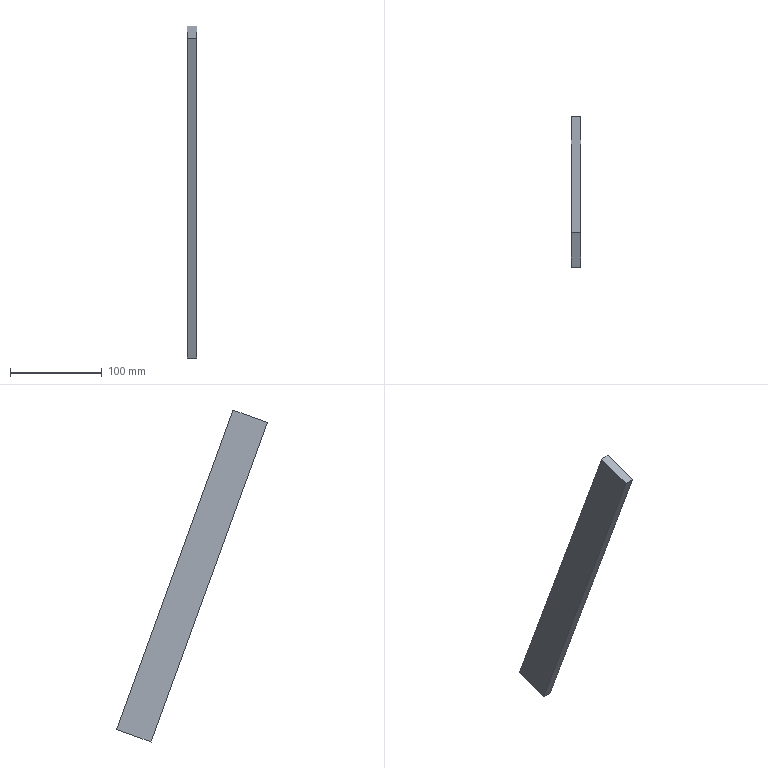Component | SolidWorks | Rebro sipke-2-34 | 1 solid | 6 faces | box 10 x 164.17 x 361.36 mm | volume 148000 mm3 | plane 6
build123d program:
from build123d import *

# Parameters (mm, degrees)
BOSS_EXTRUDE1_DEPTH = 10


with BuildPart() as part:
    # Sketch1 → Boss-Extrude1 (new body)
    with BuildSketch(Plane.XY):
        Polygon((-494.224, -762.65), (-530.101, -744.961), (-366.483, -413.104), (-330.606, -430.793), align=None)
    extrude(amount=-BOSS_EXTRUDE1_DEPTH)


solid = part.part

# Placed as in the assembly
solid = solid.moved(Location((16.4, -1316.705, 597.79), (83.762, -90, 0)))
STEP:
#1=COLOUR_RGB('',0.7922,0.8196,0.9333);
#2=FILL_AREA_STYLE_COLOUR('',#1);
#3=FILL_AREA_STYLE('',(#2));
#4=SURFACE_STYLE_FILL_AREA(#3);
#5=SURFACE_SIDE_STYLE('',(#4));
#6=SURFACE_STYLE_USAGE(.BOTH.,#5);
#7=PRESENTATION_STYLE_ASSIGNMENT((#6));
#8=CARTESIAN_POINT('',(1.039,-34.279,-7.888));
#9=VERTEX_POINT('',#8);
#10=CARTESIAN_POINT('',(1.039,-39.263,5.799));
#11=VERTEX_POINT('',#10);
#12=CARTESIAN_POINT('',(1.039,-34.279,-7.888));
#13=DIRECTION('',(-0.,-0.3421,0.9397));
#14=VECTOR('',#13,39.37);
#15=LINE('',#12,#14);
#16=EDGE_CURVE('',#9,#11,#15,.T.);
#17=ORIENTED_EDGE('',*,*,#16,.F.);
#18=CARTESIAN_POINT('',(0.6457,-34.279,-7.888));
#19=VERTEX_POINT('',#18);
#20=CARTESIAN_POINT('',(0.6457,-34.279,-7.888));
#21=DIRECTION('',(1.,-0.,0.));
#22=VECTOR('',#21,39.37);
#23=LINE('',#20,#22);
#24=EDGE_CURVE('',#19,#9,#23,.T.);
#25=ORIENTED_EDGE('',*,*,#24,.F.);
#26=CARTESIAN_POINT('',(0.6457,-39.263,5.799));
#27=VERTEX_POINT('',#26);
#28=CARTESIAN_POINT('',(0.6457,-34.279,-7.888));
#29=DIRECTION('',(-0.,-0.3421,0.9397));
#30=VECTOR('',#29,39.37);
#31=LINE('',#28,#30);
#32=EDGE_CURVE('',#19,#27,#31,.T.);
#33=ORIENTED_EDGE('',*,*,#32,.T.);
#34=CARTESIAN_POINT('',(0.6457,-39.263,5.799));
#35=DIRECTION('',(1.,-0.,0.));
#36=VECTOR('',#35,39.37);
#37=LINE('',#34,#36);
#38=EDGE_CURVE('',#27,#11,#37,.T.);
#39=ORIENTED_EDGE('',*,*,#38,.T.);
#40=EDGE_LOOP('',(#17,#25,#33,#39));
#41=FACE_OUTER_BOUND('',#40,.T.);
#42=CARTESIAN_POINT('',(0.6457,-34.279,-7.888));
#43=DIRECTION('',(0.,0.9397,0.3421));
#44=DIRECTION('',(-0.,-0.3421,0.9397));
#45=AXIS2_PLACEMENT_3D('',#42,#43,#44);
#46=PLANE('',#45);
#47=ADVANCED_FACE('',(#41),#46,.T.);
#48=CARTESIAN_POINT('',(1.039,-35.759,-8.427));
#49=VERTEX_POINT('',#48);
#50=CARTESIAN_POINT('',(1.039,-34.279,-7.888));
#51=DIRECTION('',(0.,0.9397,0.3421));
#52=VECTOR('',#51,39.37);
#53=LINE('',#50,#52);
#54=EDGE_CURVE('',#49,#9,#53,.T.);
#55=ORIENTED_EDGE('',*,*,#54,.F.);
#56=CARTESIAN_POINT('',(0.6457,-35.759,-8.427));
#57=VERTEX_POINT('',#56);
#58=CARTESIAN_POINT('',(0.6457,-35.759,-8.427));
#59=DIRECTION('',(1.,-0.,0.));
#60=VECTOR('',#59,39.37);
#61=LINE('',#58,#60);
#62=EDGE_CURVE('',#57,#49,#61,.T.);
#63=ORIENTED_EDGE('',*,*,#62,.F.);
#64=CARTESIAN_POINT('',(0.6457,-34.279,-7.888));
#65=DIRECTION('',(0.,0.9397,0.3421));
#66=VECTOR('',#65,39.37);
#67=LINE('',#64,#66);
#68=EDGE_CURVE('',#57,#19,#67,.T.);
#69=ORIENTED_EDGE('',*,*,#68,.T.);
#70=ORIENTED_EDGE('',*,*,#24,.T.);
#71=EDGE_LOOP('',(#55,#63,#69,#70));
#72=FACE_OUTER_BOUND('',#71,.T.);
#73=CARTESIAN_POINT('',(0.6457,-34.279,-7.888));
#74=DIRECTION('',(0.,0.3421,-0.9397));
#75=DIRECTION('',(0.,0.9397,0.3421));
#76=AXIS2_PLACEMENT_3D('',#73,#74,#75);
#77=PLANE('',#76);
#78=ADVANCED_FACE('',(#72),#77,.T.);
#79=CARTESIAN_POINT('',(1.039,-40.743,5.261));
#80=VERTEX_POINT('',#79);
#81=CARTESIAN_POINT('',(1.039,-35.759,-8.427));
#82=DIRECTION('',(0.,0.3421,-0.9397));
#83=VECTOR('',#82,39.37);
#84=LINE('',#81,#83);
#85=EDGE_CURVE('',#80,#49,#84,.T.);
#86=ORIENTED_EDGE('',*,*,#85,.F.);
#87=CARTESIAN_POINT('',(0.6457,-40.743,5.261));
#88=VERTEX_POINT('',#87);
#89=CARTESIAN_POINT('',(0.6457,-40.743,5.261));
#90=DIRECTION('',(1.,-0.,0.));
#91=VECTOR('',#90,39.37);
#92=LINE('',#89,#91);
#93=EDGE_CURVE('',#88,#80,#92,.T.);
#94=ORIENTED_EDGE('',*,*,#93,.F.);
#95=CARTESIAN_POINT('',(0.6457,-35.759,-8.427));
#96=DIRECTION('',(0.,0.3421,-0.9397));
#97=VECTOR('',#96,39.37);
#98=LINE('',#95,#97);
#99=EDGE_CURVE('',#88,#57,#98,.T.);
#100=ORIENTED_EDGE('',*,*,#99,.T.);
#101=ORIENTED_EDGE('',*,*,#62,.T.);
#102=EDGE_LOOP('',(#86,#94,#100,#101));
#103=FACE_OUTER_BOUND('',#102,.T.);
#104=CARTESIAN_POINT('',(0.6457,-35.759,-8.427));
#105=DIRECTION('',(-0.,-0.9397,-0.3421));
#106=DIRECTION('',(0.,0.3421,-0.9397));
#107=AXIS2_PLACEMENT_3D('',#104,#105,#106);
#108=PLANE('',#107);
#109=ADVANCED_FACE('',(#103),#108,.T.);
#110=CARTESIAN_POINT('',(1.039,-39.263,5.799));
#111=DIRECTION('',(-0.,-0.9397,-0.3421));
#112=VECTOR('',#111,39.37);
#113=LINE('',#110,#112);
#114=EDGE_CURVE('',#11,#80,#113,.T.);
#115=ORIENTED_EDGE('',*,*,#114,.F.);
#116=ORIENTED_EDGE('',*,*,#38,.F.);
#117=CARTESIAN_POINT('',(0.6457,-39.263,5.799));
#118=DIRECTION('',(-0.,-0.9397,-0.3421));
#119=VECTOR('',#118,39.37);
#120=LINE('',#117,#119);
#121=EDGE_CURVE('',#27,#88,#120,.T.);
#122=ORIENTED_EDGE('',*,*,#121,.T.);
#123=ORIENTED_EDGE('',*,*,#93,.T.);
#124=EDGE_LOOP('',(#115,#116,#122,#123));
#125=FACE_OUTER_BOUND('',#124,.T.);
#126=CARTESIAN_POINT('',(0.6457,-39.263,5.799));
#127=DIRECTION('',(-0.,-0.3421,0.9397));
#128=DIRECTION('',(-0.,-0.9397,-0.3421));
#129=AXIS2_PLACEMENT_3D('',#126,#127,#128);
#130=PLANE('',#129);
#131=ADVANCED_FACE('',(#125),#130,.T.);
#132=ORIENTED_EDGE('',*,*,#32,.F.);
#133=ORIENTED_EDGE('',*,*,#68,.F.);
#134=ORIENTED_EDGE('',*,*,#99,.F.);
#135=ORIENTED_EDGE('',*,*,#121,.F.);
#136=EDGE_LOOP('',(#132,#133,#134,#135));
#137=FACE_OUTER_BOUND('',#136,.T.);
#138=CARTESIAN_POINT('',(0.6457,-42.515,26.93));
#139=DIRECTION('',(1.,-0.,0.));
#140=DIRECTION('',(-0.,0.6915,0.7224));
#141=AXIS2_PLACEMENT_3D('',#138,#139,#140);
#142=PLANE('',#141);
#143=ADVANCED_FACE('',(#137),#142,.F.);
#144=ORIENTED_EDGE('',*,*,#16,.T.);
#145=ORIENTED_EDGE('',*,*,#114,.T.);
#146=ORIENTED_EDGE('',*,*,#85,.T.);
#147=ORIENTED_EDGE('',*,*,#54,.T.);
#148=EDGE_LOOP('',(#144,#145,#146,#147));
#149=FACE_OUTER_BOUND('',#148,.T.);
#150=CARTESIAN_POINT('',(1.039,-42.515,26.93));
#151=DIRECTION('',(1.,-0.,0.));
#152=DIRECTION('',(-0.,0.6915,0.7224));
#153=AXIS2_PLACEMENT_3D('',#150,#151,#152);
#154=PLANE('',#153);
#155=ADVANCED_FACE('',(#149),#154,.T.);
#156=CLOSED_SHELL('',(#47,#78,#109,#131,#143,#155));
#157=MANIFOLD_SOLID_BREP('',#156);
#158=STYLED_ITEM('',(#7),#157);
#159=PRESENTATION_LAYER_ASSIGNMENT('','',(#158));
#160=(LENGTH_UNIT()NAMED_UNIT(*)SI_UNIT($,.METRE.));
#161=LENGTH_MEASURE_WITH_UNIT(LENGTH_MEASURE(0.0254),#160);
#162=DIMENSIONAL_EXPONENTS(1.,0.,0.,0.,0.,0.,0.);
#163=(CONVERSION_BASED_UNIT('',#161)LENGTH_UNIT()NAMED_UNIT(#162));
#164=UNCERTAINTY_MEASURE_WITH_UNIT(LENGTH_MEASURE(0.00001),#163,'','');
#165=(NAMED_UNIT(*)PLANE_ANGLE_UNIT()SI_UNIT($,.RADIAN.));
#166=(NAMED_UNIT(*)SI_UNIT($,.STERADIAN.)SOLID_ANGLE_UNIT());
#167=(GEOMETRIC_REPRESENTATION_CONTEXT(3)GLOBAL_UNCERTAINTY_ASSIGNED_CONTEXT((#164))GLOBAL_UNIT_ASSIGNED_CONTEXT((#163,#165,#166))REPRESENTATION_CONTEXT('',''));
#168=MECHANICAL_DESIGN_GEOMETRIC_PRESENTATION_REPRESENTATION('',(#158),#167);
#169=CARTESIAN_POINT('',(0.,0.,0.));
#170=DIRECTION('',(0.,0.,1.));
#171=DIRECTION('',(1.,0.,0.));
#172=AXIS2_PLACEMENT_3D('',#169,#170,#171);
#173=(LENGTH_UNIT()NAMED_UNIT(*)SI_UNIT($,.METRE.));
#174=LENGTH_MEASURE_WITH_UNIT(LENGTH_MEASURE(0.0254),#173);
#175=DIMENSIONAL_EXPONENTS(1.,0.,0.,0.,0.,0.,0.);
#176=(CONVERSION_BASED_UNIT('',#174)LENGTH_UNIT()NAMED_UNIT(#175));
#177=UNCERTAINTY_MEASURE_WITH_UNIT(LENGTH_MEASURE(0.00001),#176,'','');
#178=(NAMED_UNIT(*)PLANE_ANGLE_UNIT()SI_UNIT($,.RADIAN.));
#179=(NAMED_UNIT(*)SI_UNIT($,.STERADIAN.)SOLID_ANGLE_UNIT());
#180=(GEOMETRIC_REPRESENTATION_CONTEXT(3)GLOBAL_UNCERTAINTY_ASSIGNED_CONTEXT((#177))GLOBAL_UNIT_ASSIGNED_CONTEXT((#176,#178,#179))REPRESENTATION_CONTEXT('',''));
#181=ADVANCED_BREP_SHAPE_REPRESENTATION('',(#157,#172),#180);